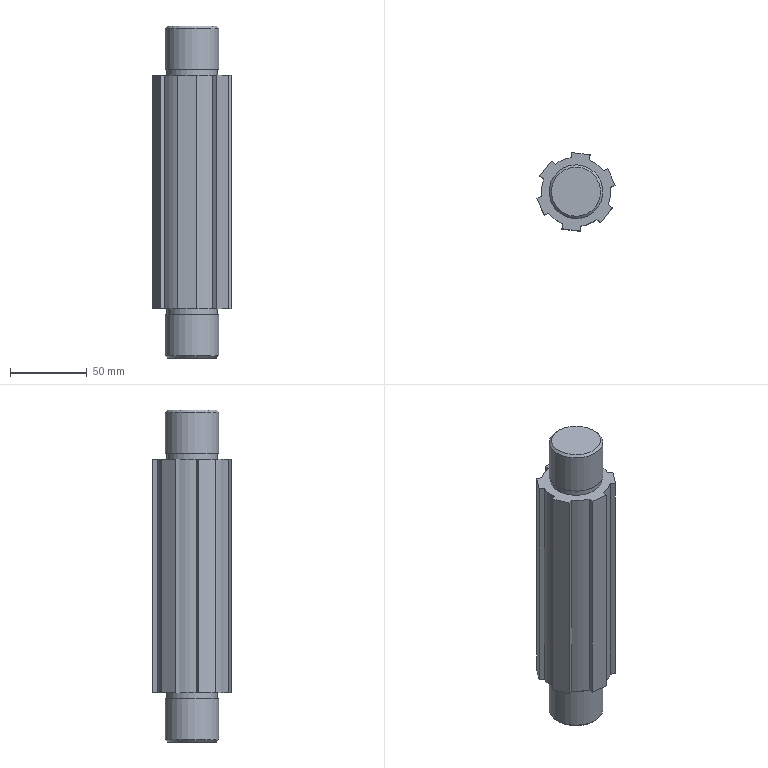Component | NX | ZHOUV1 | 1 solid | 36 faces | volume 332315 mm3 | plane 24 | cylinder 10 | cone 2 | commonest cylinder face diameters 45 x6 35 x2 33 x2